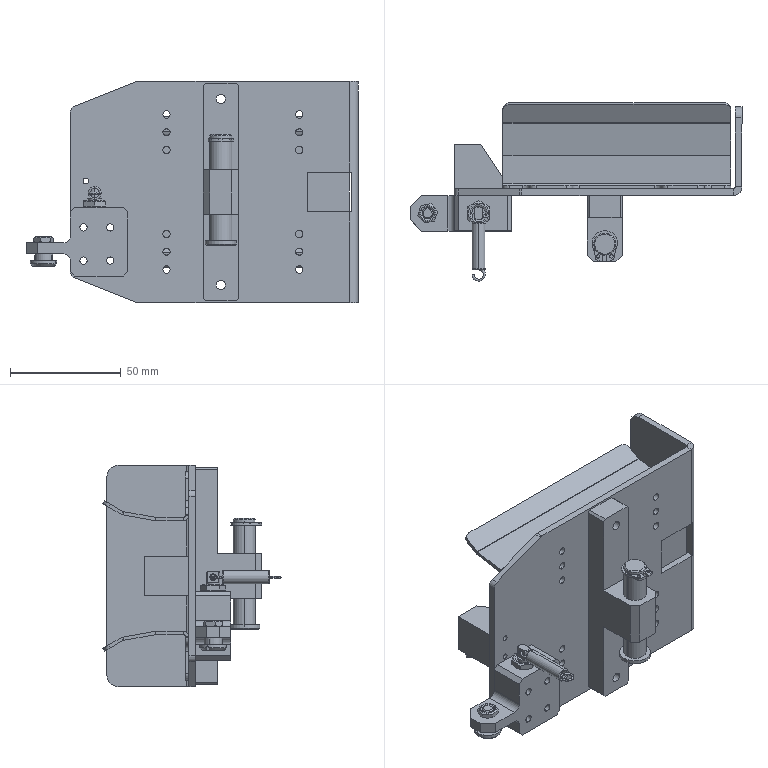Assembly | SolidWorks | mm | 14 component files | 14 solids | 407 faces | box 150 x 80.52 x 100 mm | volume 106375 mm3 | plane 191 | cylinder 173 | cone 35 | spline 8 | commonest cylinder face diameters 6 x42 3.3 x32 5 x22 4.5 x12 2 x8 10 x8 4.2 x6 9.6 x5
Bill of materials:
HexThinNutGBT6172.1-M5 | 1 | Purchased Part | Thin hexagonal nut-like ring with a central round through-bore and chamfered hex corners on both faces.
HexThinNutGBT6172.1-M6 | 1 | Purchased Part | Thin hexagonal nut-like ring with a central round through-bore and chamfered corners on both faces; very close in form to unnamed part.
RetainingRingPinMIC06_D10_L45 | 1 |  | Headed cylindrical pin: a long plain shank with a thin, wider flange head at one end and a shallow circumferential groove near the other, chamfered end.
ShaftRetainingRing_10 | 1 | Purchased Part | Flat open ring shaped like an external retaining clip: a circular band with a gap and two flared lugs, each with a small round hole.
SpringPillarFFE01-D6-L20 | 1 | Purchased Part | Cylindrical pin whose upper end is machined down to a reduced, flat-sided tenon with a transverse through-hole; the other end is chamfered.
StepScrewForFulcrumMJR06_D8_L3_A12_E2_5_F8 | 1 |  | Stepped cylindrical pin with three coaxial diameters: a chamfered small-diameter pin, a middle collar, and a wide flange base with a chamfered underside and one small radial slot or notch.
WashingLabel100-50 | 1 | Zoltek Panex 33 | Flat rectangular sheet with a single small round hole at its center; it appears to have essentially zero thickness.
XM-02-005A1 | 1 | SUS304 | Sheet-metal L-bracket: a large flat web with angled corner chamfers, bent 90 degrees into a short flange at one edge; the web carries several hole patterns.
XM-02-006A1 | 2 | SUS304 | Formed sheet-metal channel or tray: a long base bent in several shallow angles that rises into a sloped lip on one side, with two upright tabs on the other side, each with a vertical slot.
XM-02-007A1 | 1 | 45# | T-shaped block: a long, narrow rectangular bar with a small round hole near each end and a rectangular boss projecting from its middle, carrying a larger through-hole parallel to the bar's long axis.
XM-02-008A1 | 1 | Black POM | Prismatic block with one corner cut off by an angled plane, giving a pentagonal profile; two round through-holes pass through one rectangular face.
XM-02-009A1 | 1 | 45# | Rectangular block with chamfered corners and four holes in a square pattern on one face; a thinner tab with a hole and chamfered end extends from one side, and one blind conical-bottom hole sits on the top face.
YAWF-D6-L30 | 1 | Purchased Part | Elongated, smooth, hollow cylindrical body with an open, round wire hook at each end. The hooks lie in the same plane, which runs through the body axis. The shape matches a simplified extension spring with the coils modeled as a plain tube.
Mates:
1. coincident | XM-02-005A1-1 face at (0, 0, 0) dir (0, 1, 0) | XM-02-006A1-1 face at (8.5, 0, 36) dir (0, -1, 0)
2. distance | XM-02-005A1-1 face at (62, 0, 0) dir (-1, 0, 0) | XM-02-006A1-1 face at (60, 0, 47) dir (1, 0, 0)
3. coincident | XM-02-005A1-1 face at (0, 0, 0) dir (0, 1, 0) | XM-02-006A1-2 face at (8.5, 0, -36) dir (0, -1, 0)
4. coincident | XM-02-005A1-1 face at (0, 0, 0) dir (0, 1, 0) | WashingLabel100-50-1 face at (12, 0, 0) dir (0, -1, 0)
5. coincident | XM-02-006A1-2 face at (8.5, 1.5, -25) dir (0, 0, 1) | WashingLabel100-50-1 face at (62, 0.1, -25) dir (0, 0, -1)
6. coincident | XM-02-005A1-1 face at (0, -3, 0) dir (0, -1, 0) | XM-02-007A1-1 face at (11, -3, -49) dir (0, 1, 0)
7. width | XM-02-007A1-1 face at (11, -3, 49) dir (0, 0, 1) | XM-02-007A1-1 face at (11, -13, -49) dir (0, 0, -1) | XM-02-005A1-1 face at (-65, -3, -50) dir (0, 0, -1) | XM-02-005A1-1 face at (-65, -3, 50) dir (0, 0, 1)
8. distance | XM-02-007A1-1 face at (-5, -33, 0) dir (-1, 0, 0) | XM-02-005A1-1 face at (-65, -3, -50) dir (-1, 0, 0)
9. concentric | XM-02-009A1-1 face at (-77, -11, -28) dir (0, 0, -1) r 2.5 | StepScrewForFulcrumMJR06_D8_L3_A12_E2_5_F8-1 face at (-77, -11, -20) dir (0, 0, 1) r 4
10. coincident | XM-02-009A1-1 face at (-39, -19, -28) dir (0, 0, -1) | StepScrewForFulcrumMJR06_D8_L3_A12_E2_5_F8-1 face at (-75.302, -7.378, -28) dir (0, 0, 1)
11. concentric | HexThinNutGBT6172.1-M5-1 face at (-77, -11, -23) dir (0, 0, 1) r 2.5 | StepScrewForFulcrumMJR06_D8_L3_A12_E2_5_F8-1 face at (-77, -11, -20) dir (0, 0, 1) r 2.5
12. coincident | XM-02-009A1-1 face at (-39, -19, -23) dir (0, 0, 1) | HexThinNutGBT6172.1-M5-1 face at (-81.535, -11.878, -23) dir (0, 0, -1)
13. concentric | XM-02-007A1-1 face at (3, -25, 49) dir (0, 0, -1) r 5 | RetainingRingPinMIC06_D10_L45-1 face at (3, -25, 23) dir (0, 0, 1) r 5
14. distance | RetainingRingPinMIC06_D10_L45-1 face at (3, -18, -22) dir (0, 0, 1) | XM-02-007A1-1 face at (11, -33, -10) dir (0, 0, -1)
15. concentric | ShaftRetainingRing_10-1 face at (3, -25, 23) dir (0, 0, 1) r 4.8 | RetainingRingPinMIC06_D10_L45-1 face at (3, -25, 26) dir (0, 0, 1) r 4.8
16. coincident | ShaftRetainingRing_10-1 face at (3, -25, 23) dir (0, 0, -1) | RetainingRingPinMIC06_D10_L45-1 face at (3, -20, 23) dir (0, 0, 1)
17. coincident | XM-02-006A1-1 face at (-43, 15, 25) dir (-1, 0, 0) | XM-02-006A1-2 face at (-43, 1.5, -25) dir (-1, 0, 0)
18. coincident | XM-02-005A1-1 face at (0, 0, 0) dir (0, 1, 0) | XM-02-008A1-1 face at (-54, 0, 0) dir (0, -1, 0)
19. coincident | XM-02-005A1-1 face at (-65, -3, -50) dir (-1, 0, 0) | XM-02-008A1-1 face at (-65, 20, -9) dir (-1, 0, 0)
20. width | XM-02-008A1-1 face at (-43, 20, -9) dir (0, 0, -1) | XM-02-008A1-1 face at (-43, 20, 9) dir (0, 0, 1) | XM-02-005A1-1 face at (-65, -3, 50) dir (0, 0, 1) | XM-02-005A1-1 face at (-65, -3, -50) dir (0, 0, -1)
21. coincident | XM-02-005A1-1 face at (0, -3, 0) dir (0, -1, 0) | XM-02-009A1-1 face at (-39, -3, -28) dir (0, 1, 0)
22. coincident | XM-02-005A1-1 face at (-65, -3, -50) dir (-1, 0, 0) | XM-02-009A1-1 face at (-65, -3, -7) dir (-1, 0, 0)
23. distance | XM-02-009A1-1 face at (-39, -19, -28) dir (0, 0, -1) | XM-02-005A1-1 face at (-65, -3, -50) dir (0, 0, -1)
24. concentric | XM-02-009A1-1 face at (-54, -11, -7) dir (0, 0, 1) r 3 | SpringPillarFFE01-D6-L20-1 face at (-54, -11, -18) dir (0, 0, 1) r 3
25. distance | XM-02-009A1-1 face at (-39, -3, -7) dir (0, 0, 1) | SpringPillarFFE01-D6-L20-1 face at (-55.75, -8, -3) dir (0, 0, 1)
26. parallel | XM-02-009A1-1 face at (-65, -3, -7) dir (-1, 0, 0) | SpringPillarFFE01-D6-L20-1 face at (-55.75, -8, 2) dir (-1, 0, 0)
27. distance | YAWF-D6-L30-1 plane at (-53.95, -15, -0.5) dir (1, 0, 0) | SpringPillarFFE01-D6-L20-1 face at (-55.75, -8, 2) dir (-1, 0, 0)
28. distance | YAWF-D6-L30-1 plane at (-53.95, -15, -0.5) dir (0, 0, 1) | SpringPillarFFE01-D6-L20-1 face at (-54, -11, 2) dir (0, 0, 1)
29. distance | YAWF-D6-L30-1 plane at (-53.95, -15, -0.5) dir (0, 1, 0) | SpringPillarFFE01-D6-L20-1 plane at (-54, -11, 2) dir (0, 1, 0)
30. distance | XM-02-006A1-1 face at (8.5, 1.5, 25) dir (0, 0, -1) | XM-02-005A1-1 face at (-65, -3, 50) dir (0, 0, 1)
31. distance | XM-02-006A1-2 face at (8.5, 1.5, -25) dir (0, 0, 1) | XM-02-005A1-1 face at (-65, -3, -50) dir (0, 0, -1)
32. concentric | SpringPillarFFE01-D6-L20-1 face at (-54, -11, -18) dir (0, 0, 1) r 3 | HexThinNutGBT6172.1-M6-1 face at (-54, -11, -7) dir (0, 0, 1) r 3
33. coincident | XM-02-009A1-1 face at (-39, -3, -7) dir (0, 0, 1) | HexThinNutGBT6172.1-M6-1 face at (-54.003, -16.774, -7) dir (0, 0, -1)
34. distance | XM-02-005A1-1 face at (62, 0, 0) dir (-1, 0, 0) | WashingLabel100-50-1 face at (61, 0.1, -25) dir (1, 0, 0)